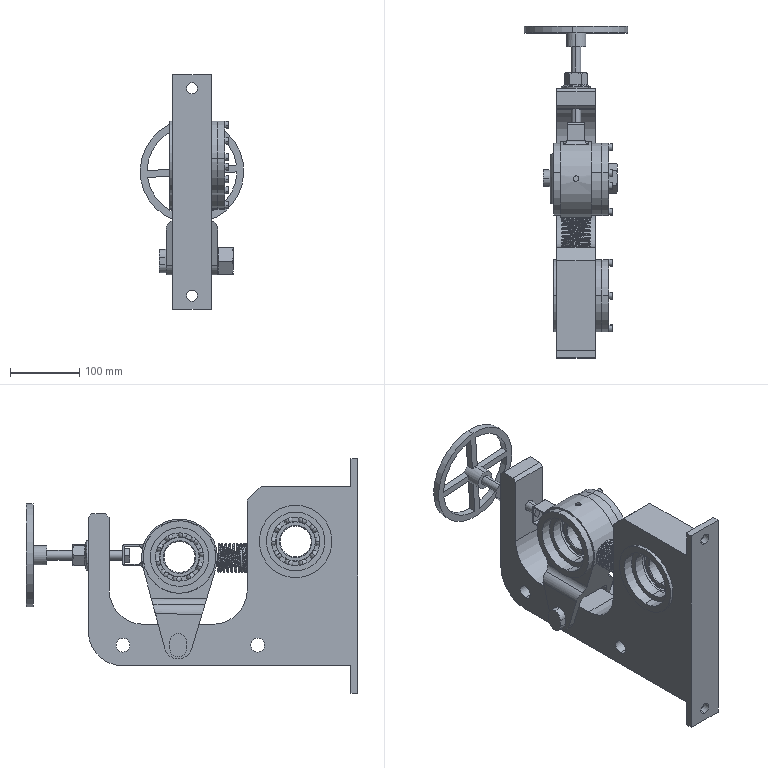Assembly | SolidWorks | mm | 24 component files | 46 solids | 664 faces | box 150 x 480 x 340 mm | volume 4059482 mm3 | plane 234 | cylinder 215 | torus 84 | cone 78 | sphere 40 | spline 13 | commonest cylinder face diameters 6 x48 20 x38 10 x23 85 x16 105 x12 70 x8 57.6 x8 45 x8
Bill of materials:
adjuster roll | 1 |  | Spoked handwheel: thin circular rim with four straight spokes meeting at a central cylindrical hub, with a long slender round shaft sticking out of one side of the hub and ending in a short hexagonal head.
penahan bearing | 2 |  | Thin-walled, short, plain cylindrical ring or sleeve with square-cut ends.
rumah bearing | 2 | ASTM A36 Steel | Thick-walled cylindrical tube or sleeve with an open through bore. Four small holes are spaced evenly around one annular end face.
SKF_6209 | 2 |  | Ring-shaped rolling-element assembly that looks like a single-row ball bearing: outer ring, inner ring, and a single row of ten spherical balls between them. No cage or shields are visible.
socket head cap screw_iso_M6x20 | 8 |  | Socket head cap screw-like part: a plain cylindrical shank with a chamfered free end, joined to a larger-diameter cylindrical head that has a hexagonal socket recess in its top face.
dudukan | 1 | ASTM A36 Steel | Flat plate bracket of uniform thickness with an irregular outline: a raised block region with a large round through hole, and a U-shaped cutout with filleted corners that leaves an upright arm. One edge has a perpendicular strip flange with a hole near each end. Several small holes run through the plate.
dudukan2 | 1 | ASTM A36 Steel | Clamp or strap bracket: a thin-walled cylindrical band that narrows into a tapered tab with a rounded end and a single round eye. Seen from the side, the band splits into two parallel forked legs. A small hollow square tab sticks out from the side of the ring, and a small hole sits in the top of the band.
hex flange nut gradea_iso | 1 |  | Flange nut: a hexagonal body with an integral, wider, round flange with rounded edges at one end, and a central round through bore.
hex thin nut chamfered gradeab_iso | 1 |  | Hex nut: a hexagonal prism with a central round bore and chamfered corners on both faces.
Part10 | 1 | ASTM A36 Steel | Flat annular plate (flange ring or gasket-like disk) with a large central hole and four small through holes spaced evenly near the outer edge, at the top, bottom, left, and right.
Part9 | 1 | ASTM A36 Steel | Flat annular plate with a large central hole and four small through holes near the outer edge. The holes form a pattern rotated away from the vertical and horizontal axes.
pengunci | 1 |  | Headed pin or bolt: a long round shank with an external thread at the far end, and a short head whose outline is a stadium (obround) shape with two flats.
spring2 | 1 |  | Helical coil spring made of round wire, cylindrical, with open, evenly spaced coils and plainly cut wire ends.
spring3 | 1 |  | Open-pitch cylindrical helical coil made from round-section wire, with a constant coil diameter, roughly 9-10 evenly spaced turns, and plain flat-cut wire ends. The shape matches a helical coil spring.
Mates:
1. concentric | dudukan-1 face at (-27.5, 60, -110) dir (1, 0, 0) r 10 | dudukan2-1 face at (-37.5, 60, -110) dir (1, 0, 0) r 10
2. coincident | dudukan-1 face at (27.5, 0, 0) dir (1, 0, 0) | dudukan2-1 face at (27.5, 3.354, -65.189) dir (-1, 0, 0)
3. concentric | dudukan-1 face at (-27.5, -110, 40) dir (1, 0, 0) r 52.5 | bearing dan rumahan assembly-1/rumah bearing-1 face at (-32.5, -110, 40) dir (1, 0, 0) r 52.5
4. distance | bearing dan rumahan assembly-1/rumah bearing-1 face at (37.5, -110, 40) dir (1, 0, 0) | dudukan-1 face at (27.5, 0, 0) dir (1, 0, 0)
5. concentric | dudukan2-1 face at (-37.5, 58.078, 17.486) dir (1, 0, 0) r 52.5 | bearing dan rumahan assembly-2/rumah bearing-1 face at (-32.5, 58.078, 17.486) dir (1, 0, 0) r 52.5
6. distance | bearing dan rumahan assembly-2/rumah bearing-1 face at (37.5, 58.078, 17.486) dir (1, 0, 0) | dudukan2-1 face at (22.5, 3.304, -50.189) dir (1, 0, 0)
7. concentric | dudukan-1 face at (-27.5, 60, -110) dir (1, 0, 0) r 10 | pengunci-3 face at (56.5, 60, -110) dir (-1, 0, 0) r 10
8. coincident | dudukan2-1 face at (-37.5, 58.078, 17.486) dir (-1, 0, 0) | pengunci-3 face at (-37.5, 60, -105) dir (1, 0, 0)
9. concentric | pengunci-3 face at (56.5, 60, -110) dir (-1, 0, 0) r 10 | hex thin nut chamfered gradeab_iso-1 face at (37.5, 60, -110) dir (1, 0, 0) r 11.113
10. coincident | dudukan2-1 face at (37.5, 58.078, 17.486) dir (1, 0, 0) | hex thin nut chamfered gradeab_iso-1 face at (37.5, 60, -71.9) dir (-1, 0, 0)
11. coincident | dudukan-1 face at (-27.5, -40, 0) dir (0, 1, 0) | spring2-1 face at (-0.6085, -40, 16.211) dir (0, -1, 0)
12. tangent | dudukan-1 face at (0, -30, 15.416) dir (0, -1, 0) r 15 | spring2-1 face at (-8.38, -40, 4.566) dir (1, 0, 0)
13. coincident | dudukan-1 face at (-27.5, -40, 0) dir (0, 1, 0) | spring3-1 face at (-0.02362, -40, 15.919) dir (0, -1, 0)
14. concentric | dudukan-1 face at (0, -200.001, 20) dir (0, 1, 0) r 8 | adjuster roll-1 face at (0, 250, 20) dir (0, -1, 0) r 7
15. concentric | adjuster roll-1 face at (0, 250, 20) dir (0, -1, 0) r 7 | hex flange nut gradea_iso-3 face at (0, 187.492, 20) dir (0, 1, 0) r 10
16. coincident | dudukan-1 face at (-27.5, 190, 0) dir (0, 1, 0) | hex flange nut gradea_iso-3 face at (-25.115, 190, 3.592) dir (0, -1, 0)
17. coincident | dudukan2-1 face at (-37.5, 138, 7) dir (0, -1, 0) | adjuster roll-1 face at (0, 138, 20) dir (0, 1, 0)
18. concentric | rumah bearing-1 face at (-30, 0, 0) dir (1, 0, 0) r 42.5 | penahan bearing-1 face at (40, 0, 0) dir (-1, 0, 0) r 42.5
19. concentric | rumah bearing-1 face at (-30, 0, 0) dir (1, 0, 0) r 42.5 | SKF_6209-3 face at (50, 0, 0) dir (-1, 0, 0) r 42.5
20. coincident | rumah bearing-1 face at (0, 0, 0) dir (1, 0, 0) | SKF_6209-3 face at (0, 28.433, 0) dir (-1, 0, 0)